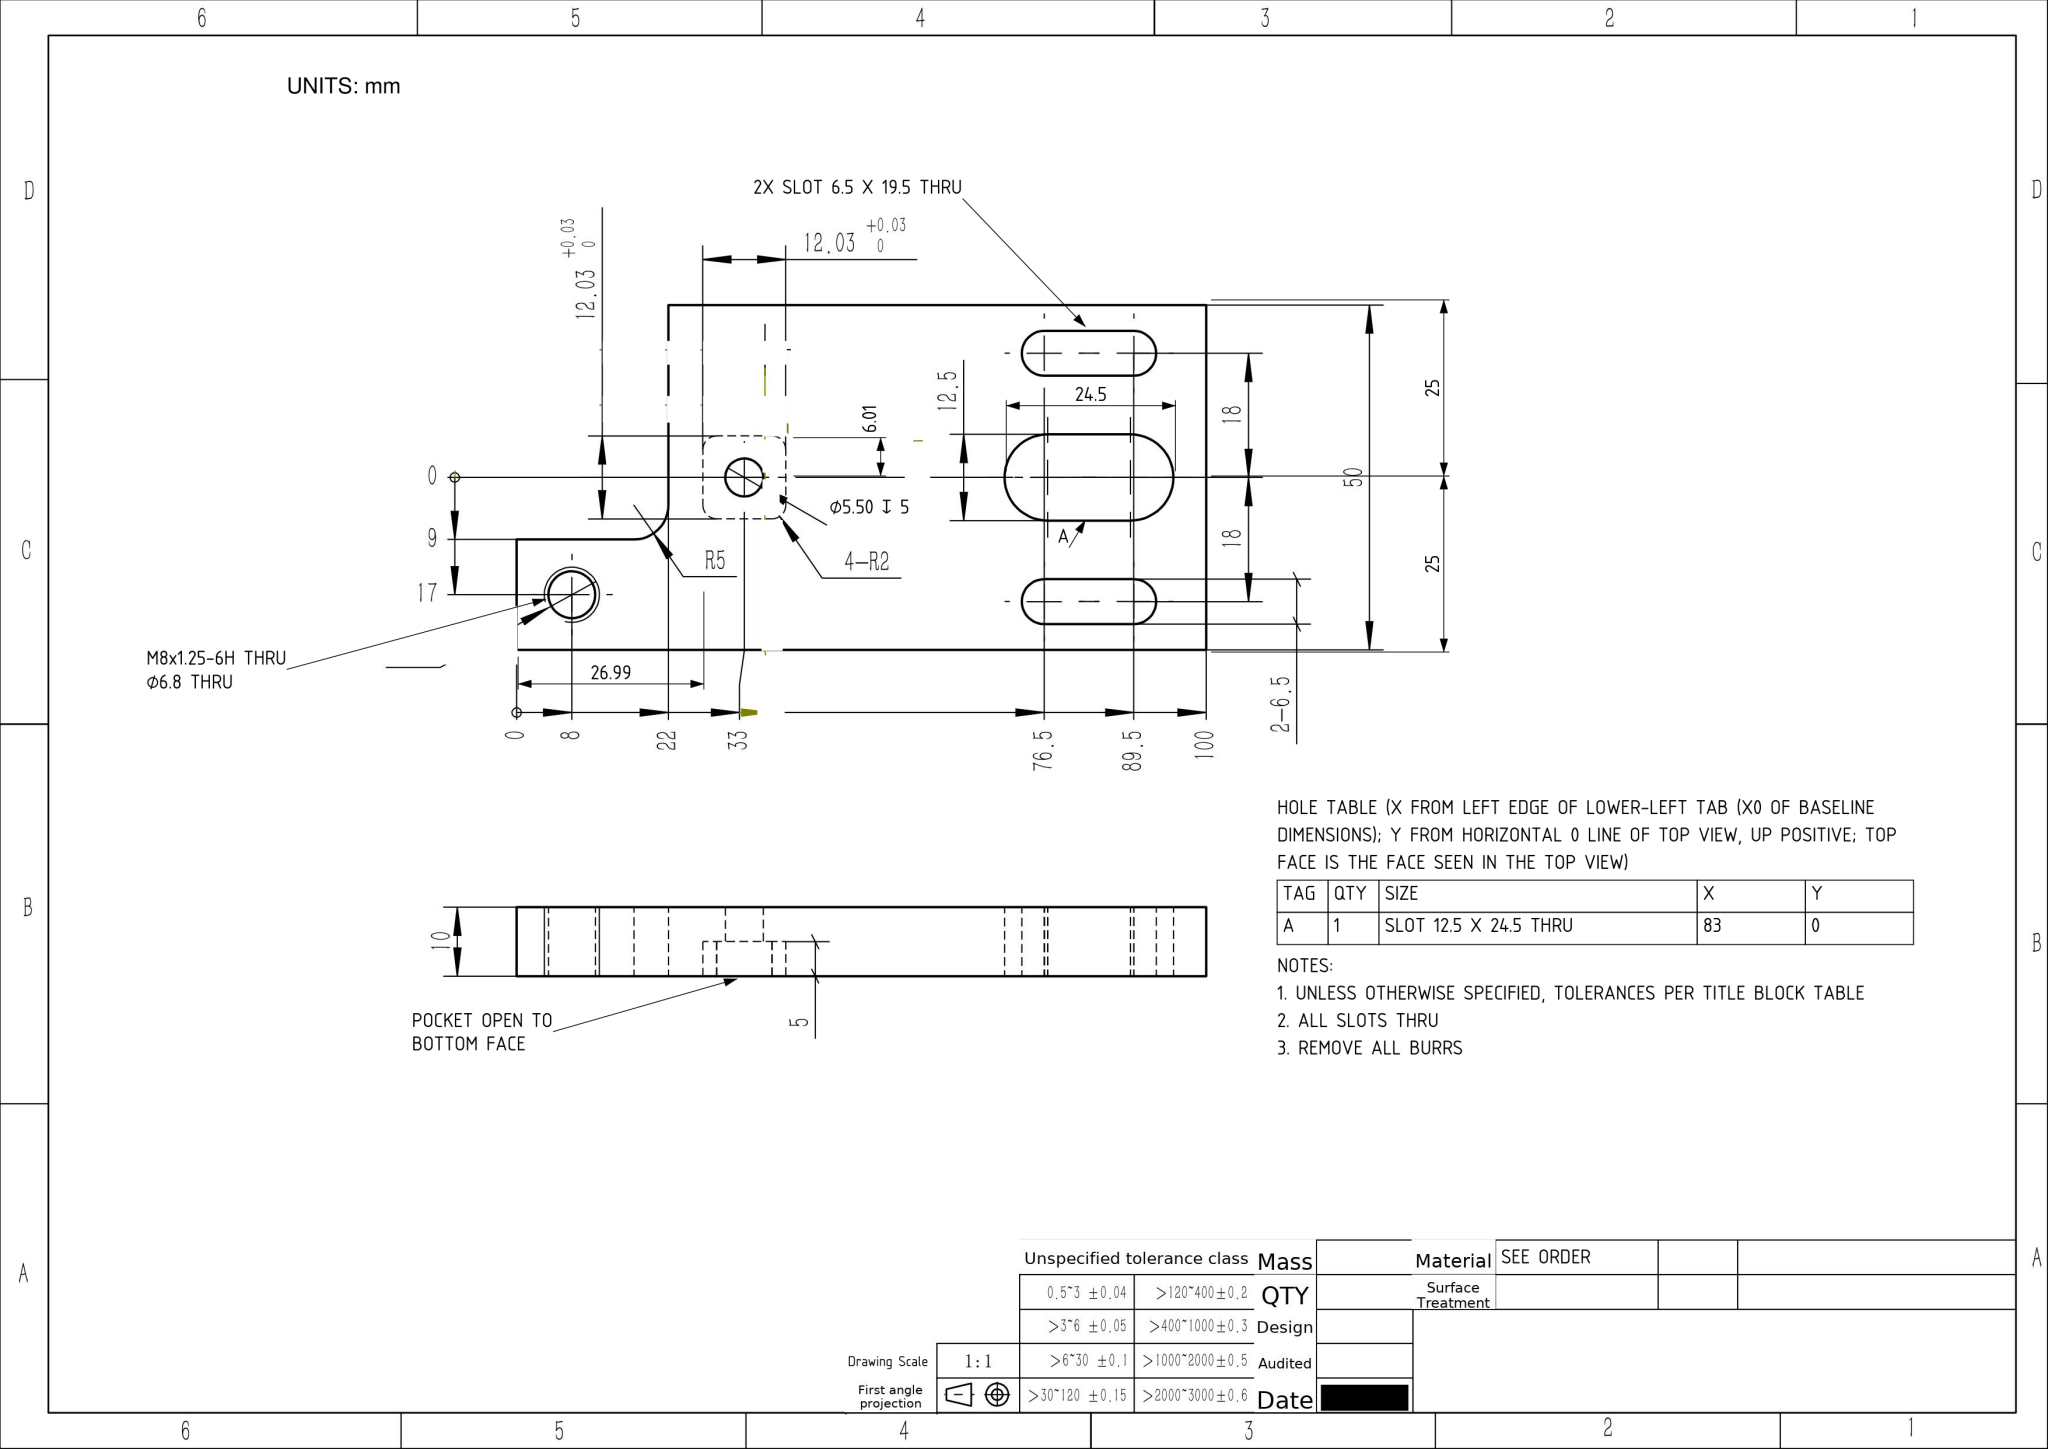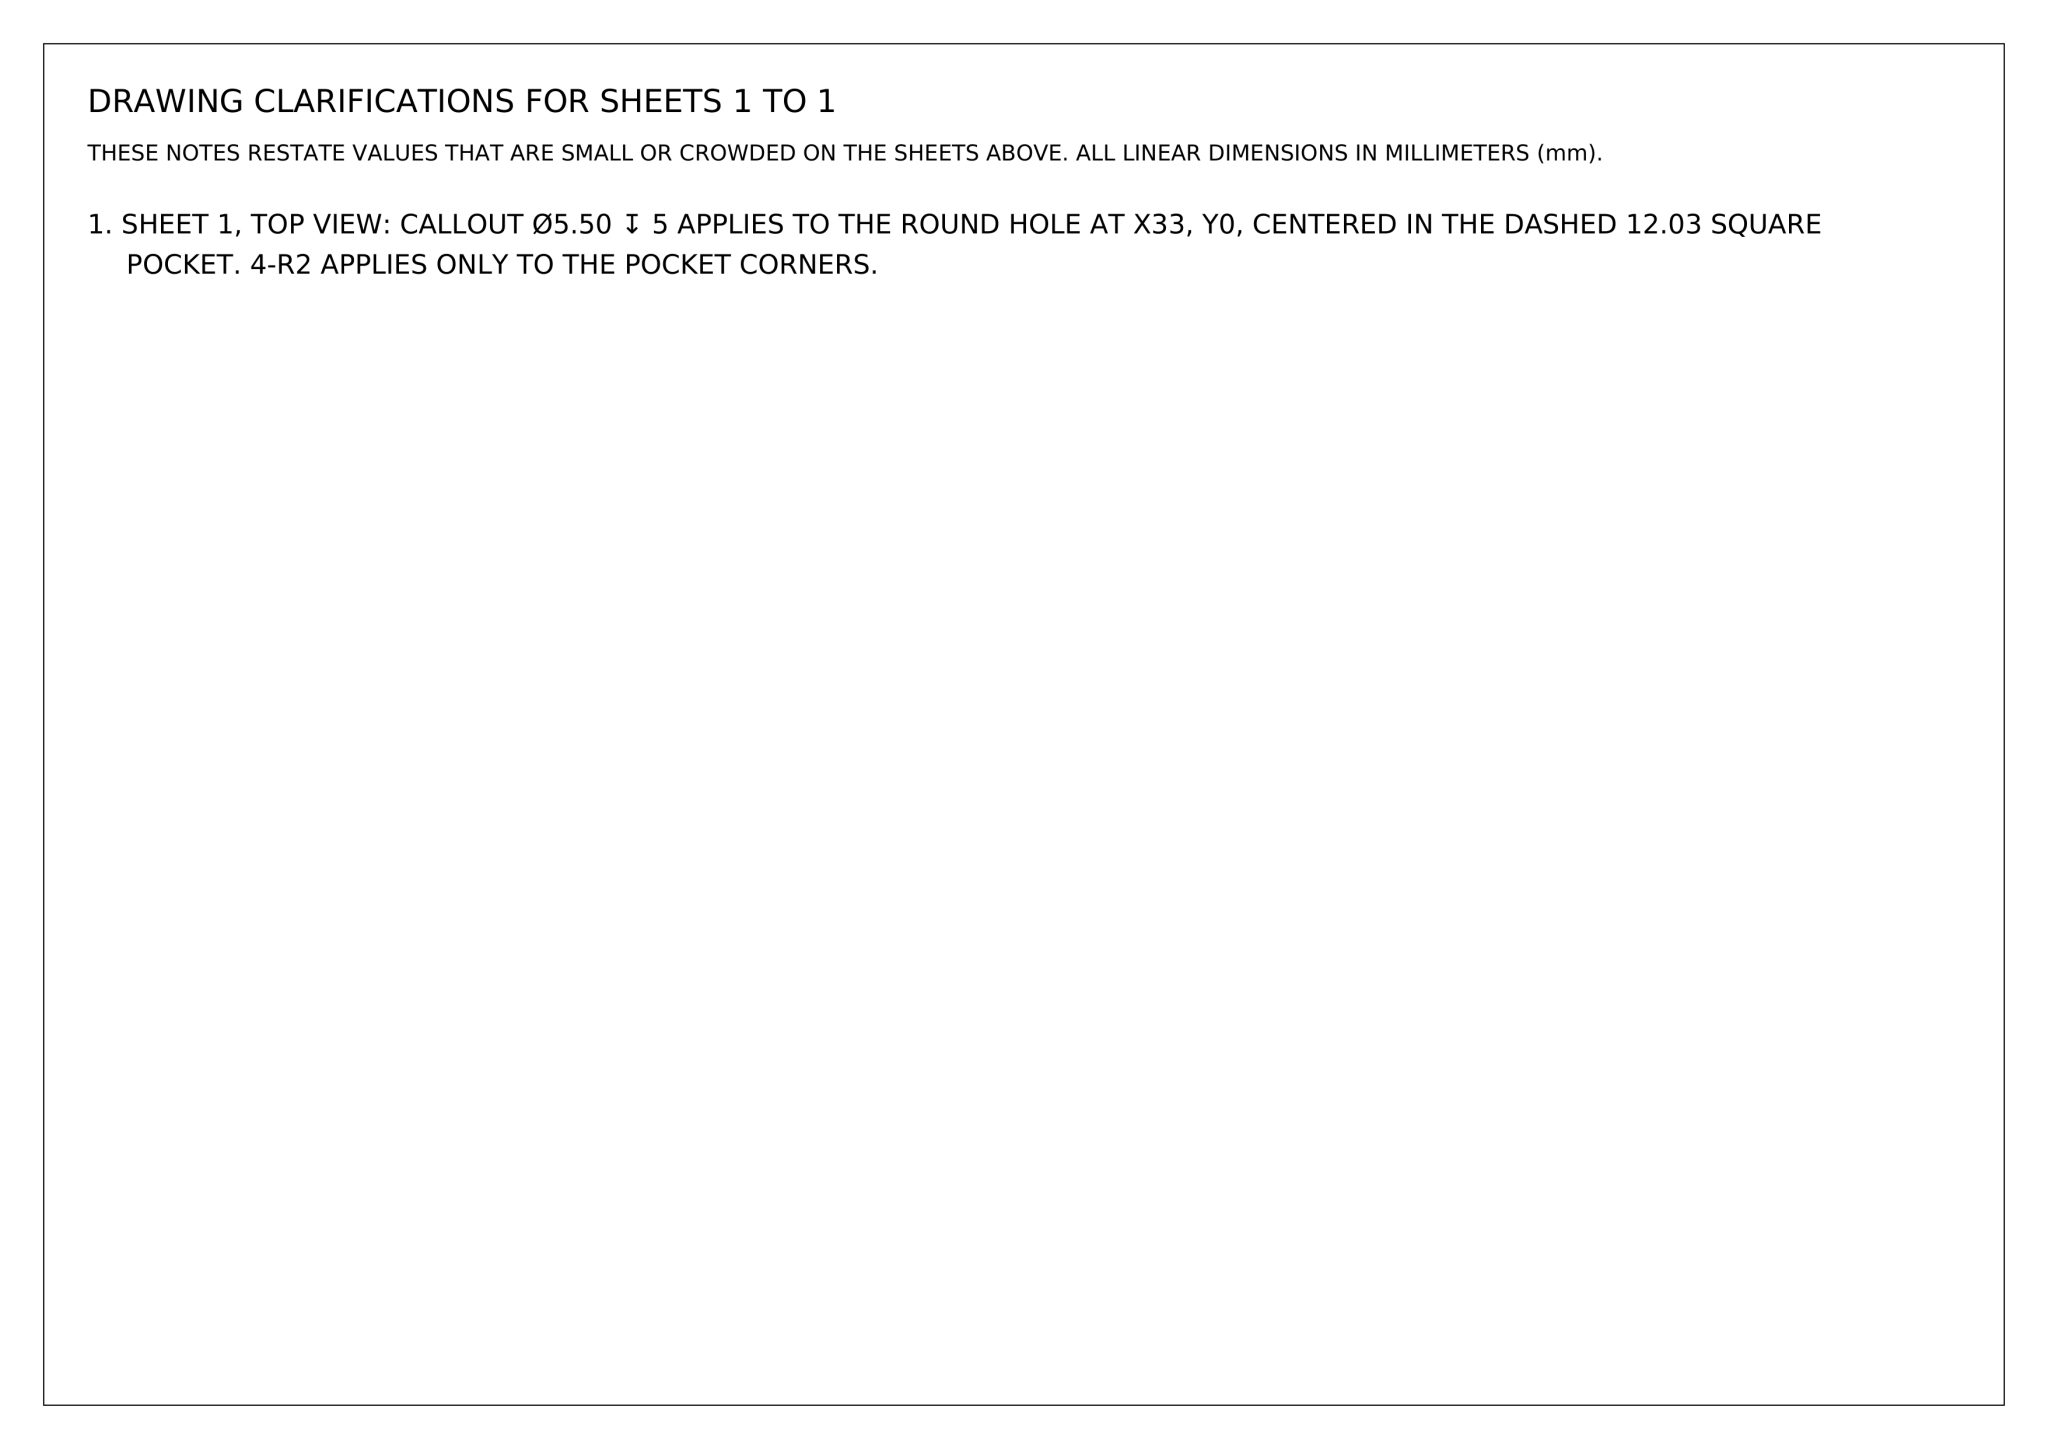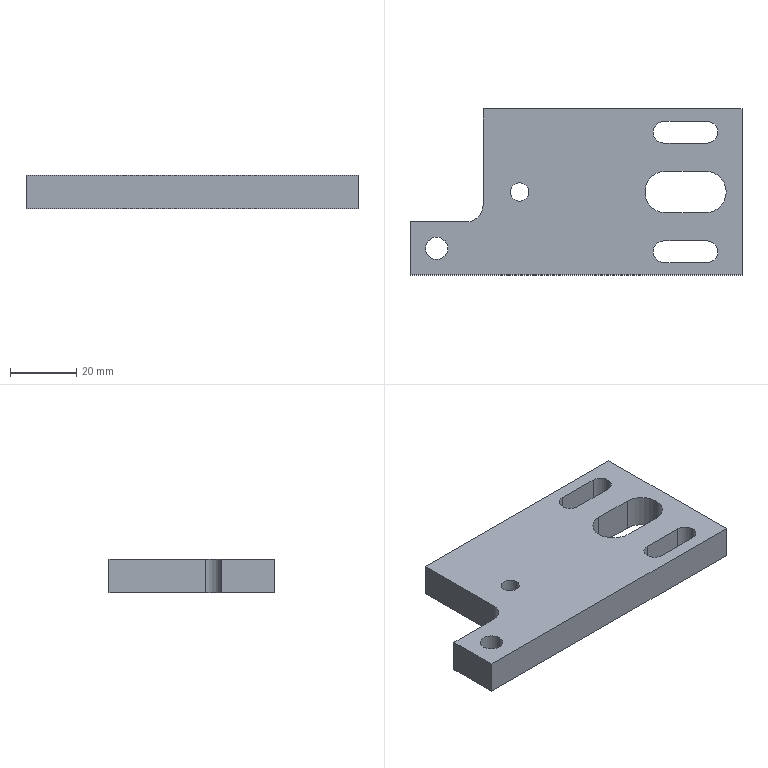Part | NX | mm | 1 solid | 37 faces | box 100 x 50 x 10 mm | volume 36304 mm3 | plane 19 | cylinder 18 | commonest cylinder face diameters 6.5 x6 4 x4 12.5 x3 6.8 x2 5.5 x2 10 x1